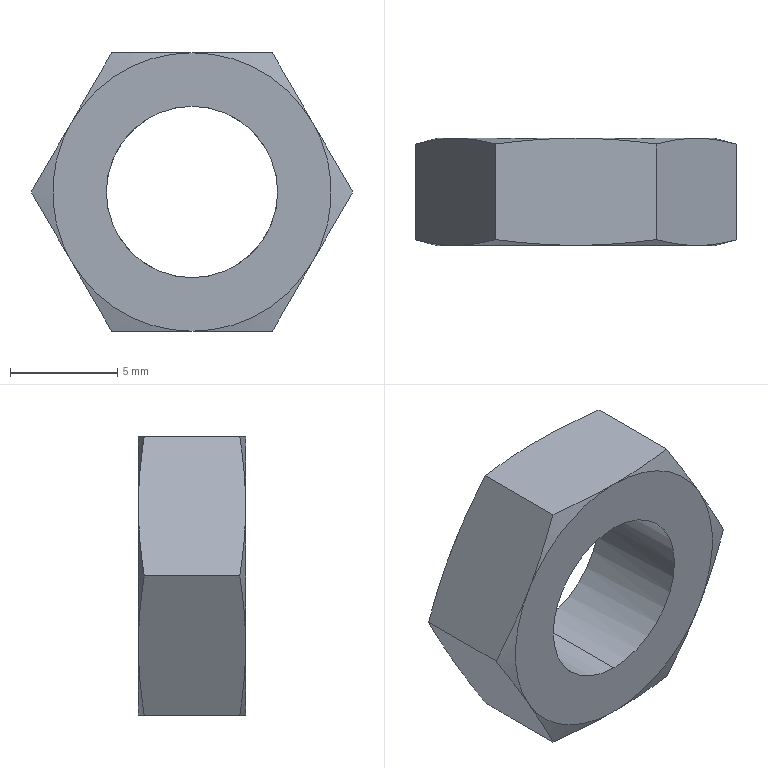Component | SolidWorks | HandlingMechanism-2_CDU25-40A-A93(0_0)-2_4..050.63-1 | 1 solid | 22 faces | box 15.01 x 5 x 13 mm | volume 478 mm3 | cone 12 | plane 8 | cylinder 2 | commonest cylinder face diameters 8 x2
STEP:
#1=CARTESIAN_POINT('',(1.019,4.705,5.787));
#2=VERTEX_POINT('',#1);
#3=CARTESIAN_POINT('',(1.019,4.705,6.102));
#4=VERTEX_POINT('',#3);
#5=CARTESIAN_POINT('',(1.019,4.705,5.945));
#6=DIRECTION('',(0.,1.,-0.));
#7=DIRECTION('',(0.,0.,1.));
#8=AXIS2_PLACEMENT_3D('',#5,#6,#7);
#9=CIRCLE('',#8,0.1575);
#10=EDGE_CURVE('',#2,#4,#9,.T.);
#11=ORIENTED_EDGE('',*,*,#10,.F.);
#12=CARTESIAN_POINT('',(1.019,4.902,5.787));
#13=VERTEX_POINT('',#12);
#14=CARTESIAN_POINT('',(1.019,4.705,5.787));
#15=DIRECTION('',(0.,1.,-0.));
#16=VECTOR('',#15,39.37);
#17=LINE('',#14,#16);
#18=EDGE_CURVE('',#2,#13,#17,.T.);
#19=ORIENTED_EDGE('',*,*,#18,.T.);
#20=CARTESIAN_POINT('',(1.019,4.902,6.102));
#21=VERTEX_POINT('',#20);
#22=CARTESIAN_POINT('',(1.019,4.902,5.787));
#23=CARTESIAN_POINT('',(0.9983,4.902,5.787));
#24=CARTESIAN_POINT('',(0.9777,4.902,5.792));
#25=CARTESIAN_POINT('',(0.9396,4.902,5.807));
#26=CARTESIAN_POINT('',(0.9221,4.902,5.819));
#27=CARTESIAN_POINT('',(0.893,4.902,5.848));
#28=CARTESIAN_POINT('',(0.8813,4.902,5.866));
#29=CARTESIAN_POINT('',(0.8655,4.902,5.904));
#30=CARTESIAN_POINT('',(0.8614,4.902,5.924));
#31=CARTESIAN_POINT('',(0.8614,4.902,5.965));
#32=CARTESIAN_POINT('',(0.8655,4.902,5.986));
#33=CARTESIAN_POINT('',(0.8813,4.902,6.024));
#34=CARTESIAN_POINT('',(0.893,4.902,6.042));
#35=CARTESIAN_POINT('',(0.9221,4.902,6.071));
#36=CARTESIAN_POINT('',(0.9396,4.902,6.082));
#37=CARTESIAN_POINT('',(0.9777,4.902,6.098));
#38=CARTESIAN_POINT('',(0.9983,4.902,6.102));
#39=CARTESIAN_POINT('',(1.019,4.902,6.102));
#40=B_SPLINE_CURVE_WITH_KNOTS('',3,(#22,#23,#24,#25,#26,#27,#28,#29,#30,#31,#32,#33,#34,#35,#36,#37,#38,#39),.UNSPECIFIED.,.F.,.F.,(4,2,2,2,2,2,2,2,4),(0.5,0.5625,0.625,0.6875,0.75,0.8125,0.875,0.9375,1.),.UNSPECIFIED.);
#41=EDGE_CURVE('',#13,#21,#40,.T.);
#42=ORIENTED_EDGE('',*,*,#41,.T.);
#43=CARTESIAN_POINT('',(1.019,4.705,6.102));
#44=DIRECTION('',(0.,1.,-0.));
#45=VECTOR('',#44,39.37);
#46=LINE('',#43,#45);
#47=EDGE_CURVE('',#4,#21,#46,.T.);
#48=ORIENTED_EDGE('',*,*,#47,.F.);
#49=EDGE_LOOP('',(#11,#19,#42,#48));
#50=FACE_OUTER_BOUND('',#49,.T.);
#51=CARTESIAN_POINT('',(1.019,4.705,5.945));
#52=DIRECTION('',(0.,1.,-0.));
#53=DIRECTION('',(0.,0.,1.));
#54=AXIS2_PLACEMENT_3D('',#51,#52,#53);
#55=CYLINDRICAL_SURFACE('',#54,0.1575);
#56=ADVANCED_FACE('',(#50),#55,.F.);
#57=CARTESIAN_POINT('',(1.019,4.705,5.945));
#58=DIRECTION('',(0.,1.,-0.));
#59=DIRECTION('',(0.,0.,1.));
#60=AXIS2_PLACEMENT_3D('',#57,#58,#59);
#61=CIRCLE('',#60,0.1575);
#62=EDGE_CURVE('',#4,#2,#61,.T.);
#63=ORIENTED_EDGE('',*,*,#62,.T.);
#64=ORIENTED_EDGE('',*,*,#10,.T.);
#65=EDGE_LOOP('',(#63,#64));
#66=FACE_BOUND('',#65,.T.);
#67=CARTESIAN_POINT('',(1.019,4.705,5.689));
#68=VERTEX_POINT('',#67);
#69=CARTESIAN_POINT('',(1.241,4.705,5.817));
#70=VERTEX_POINT('',#69);
#71=CARTESIAN_POINT('',(1.019,4.705,5.945));
#72=DIRECTION('',(-0.,-1.,0.));
#73=DIRECTION('',(0.,0.,1.));
#74=AXIS2_PLACEMENT_3D('',#71,#72,#73);
#75=CIRCLE('',#74,0.2559);
#76=EDGE_CURVE('',#68,#70,#75,.T.);
#77=ORIENTED_EDGE('',*,*,#76,.T.);
#78=CARTESIAN_POINT('',(1.241,4.705,6.073));
#79=VERTEX_POINT('',#78);
#80=CARTESIAN_POINT('',(1.019,4.705,5.945));
#81=DIRECTION('',(-0.,-1.,0.));
#82=DIRECTION('',(-0.,0.,1.));
#83=AXIS2_PLACEMENT_3D('',#80,#81,#82);
#84=CIRCLE('',#83,0.2559);
#85=EDGE_CURVE('',#70,#79,#84,.T.);
#86=ORIENTED_EDGE('',*,*,#85,.T.);
#87=CARTESIAN_POINT('',(1.019,4.705,6.201));
#88=VERTEX_POINT('',#87);
#89=CARTESIAN_POINT('',(1.019,4.705,5.945));
#90=DIRECTION('',(-0.,-1.,0.));
#91=DIRECTION('',(0.,0.,1.));
#92=AXIS2_PLACEMENT_3D('',#89,#90,#91);
#93=CIRCLE('',#92,0.2559);
#94=EDGE_CURVE('',#79,#88,#93,.T.);
#95=ORIENTED_EDGE('',*,*,#94,.T.);
#96=CARTESIAN_POINT('',(0.7973,4.705,6.073));
#97=VERTEX_POINT('',#96);
#98=CARTESIAN_POINT('',(1.019,4.705,5.945));
#99=DIRECTION('',(-0.,-1.,0.));
#100=DIRECTION('',(0.,0.,1.));
#101=AXIS2_PLACEMENT_3D('',#98,#99,#100);
#102=CIRCLE('',#101,0.2559);
#103=EDGE_CURVE('',#88,#97,#102,.T.);
#104=ORIENTED_EDGE('',*,*,#103,.T.);
#105=CARTESIAN_POINT('',(0.7973,4.705,5.817));
#106=VERTEX_POINT('',#105);
#107=CARTESIAN_POINT('',(1.019,4.705,5.945));
#108=DIRECTION('',(-0.,-1.,0.));
#109=DIRECTION('',(-0.,0.,1.));
#110=AXIS2_PLACEMENT_3D('',#107,#108,#109);
#111=CIRCLE('',#110,0.2559);
#112=EDGE_CURVE('',#97,#106,#111,.T.);
#113=ORIENTED_EDGE('',*,*,#112,.T.);
#114=CARTESIAN_POINT('',(1.019,4.705,5.945));
#115=DIRECTION('',(-0.,-1.,0.));
#116=DIRECTION('',(0.,0.,1.));
#117=AXIS2_PLACEMENT_3D('',#114,#115,#116);
#118=CIRCLE('',#117,0.2559);
#119=EDGE_CURVE('',#106,#68,#118,.T.);
#120=ORIENTED_EDGE('',*,*,#119,.T.);
#121=EDGE_LOOP('',(#77,#86,#95,#104,#113,#120));
#122=FACE_OUTER_BOUND('',#121,.T.);
#123=CARTESIAN_POINT('',(1.226,4.705,5.945));
#124=DIRECTION('',(-0.,-1.,-0.));
#125=DIRECTION('',(-0.,0.,-1.));
#126=AXIS2_PLACEMENT_3D('',#123,#124,#125);
#127=PLANE('',#126);
#128=ADVANCED_FACE('',(#66,#122),#127,.T.);
#129=ORIENTED_EDGE('',*,*,#85,.F.);
#130=CARTESIAN_POINT('',(1.314,4.715,5.945));
#131=VERTEX_POINT('',#130);
#132=CARTESIAN_POINT('',(1.241,4.705,5.817));
#133=CARTESIAN_POINT('',(1.265,4.705,5.86));
#134=CARTESIAN_POINT('',(1.29,4.709,5.902));
#135=CARTESIAN_POINT('',(1.314,4.715,5.945));
#136=B_SPLINE_CURVE_WITH_KNOTS('',3,(#132,#133,#134,#135),.UNSPECIFIED.,.F.,.F.,(4,4),(0.,0.003762),.UNSPECIFIED.);
#137=EDGE_CURVE('',#70,#131,#136,.T.);
#138=ORIENTED_EDGE('',*,*,#137,.T.);
#139=CARTESIAN_POINT('',(1.314,4.715,5.945));
#140=CARTESIAN_POINT('',(1.29,4.709,5.987));
#141=CARTESIAN_POINT('',(1.265,4.705,6.03));
#142=CARTESIAN_POINT('',(1.241,4.705,6.073));
#143=B_SPLINE_CURVE_WITH_KNOTS('',3,(#139,#140,#141,#142),.UNSPECIFIED.,.F.,.F.,(4,4),(0.,0.003762),.UNSPECIFIED.);
#144=EDGE_CURVE('',#131,#79,#143,.T.);
#145=ORIENTED_EDGE('',*,*,#144,.T.);
#146=EDGE_LOOP('',(#129,#138,#145));
#147=FACE_OUTER_BOUND('',#146,.T.);
#148=CARTESIAN_POINT('',(1.019,4.715,5.945));
#149=DIRECTION('',(0.,1.,-0.));
#150=DIRECTION('',(0.,0.,1.));
#151=AXIS2_PLACEMENT_3D('',#148,#149,#150);
#152=CONICAL_SURFACE('',#151,0.2957,1.309);
#153=ADVANCED_FACE('',(#147),#152,.T.);
#154=CARTESIAN_POINT('',(1.167,4.715,5.689));
#155=VERTEX_POINT('',#154);
#156=CARTESIAN_POINT('',(1.167,4.715,5.689));
#157=CARTESIAN_POINT('',(1.191,4.709,5.731));
#158=CARTESIAN_POINT('',(1.216,4.705,5.774));
#159=CARTESIAN_POINT('',(1.241,4.705,5.817));
#160=B_SPLINE_CURVE_WITH_KNOTS('',3,(#156,#157,#158,#159),.UNSPECIFIED.,.F.,.F.,(4,4),(0.,0.003762),.UNSPECIFIED.);
#161=EDGE_CURVE('',#155,#70,#160,.T.);
#162=ORIENTED_EDGE('',*,*,#161,.T.);
#163=ORIENTED_EDGE('',*,*,#76,.F.);
#164=CARTESIAN_POINT('',(1.019,4.705,5.689));
#165=CARTESIAN_POINT('',(1.068,4.705,5.689));
#166=CARTESIAN_POINT('',(1.118,4.709,5.689));
#167=CARTESIAN_POINT('',(1.167,4.715,5.689));
#168=B_SPLINE_CURVE_WITH_KNOTS('',3,(#164,#165,#166,#167),.UNSPECIFIED.,.F.,.F.,(4,4),(0.,0.003762),.UNSPECIFIED.);
#169=EDGE_CURVE('',#68,#155,#168,.T.);
#170=ORIENTED_EDGE('',*,*,#169,.T.);
#171=EDGE_LOOP('',(#162,#163,#170));
#172=FACE_OUTER_BOUND('',#171,.T.);
#173=CARTESIAN_POINT('',(1.019,4.715,5.945));
#174=DIRECTION('',(0.,1.,-0.));
#175=DIRECTION('',(0.,0.,1.));
#176=AXIS2_PLACEMENT_3D('',#173,#174,#175);
#177=CONICAL_SURFACE('',#176,0.2957,1.309);
#178=ADVANCED_FACE('',(#172),#177,.T.);
#179=CARTESIAN_POINT('',(0.8712,4.715,5.689));
#180=VERTEX_POINT('',#179);
#181=CARTESIAN_POINT('',(0.8712,4.715,5.689));
#182=CARTESIAN_POINT('',(0.9202,4.709,5.689));
#183=CARTESIAN_POINT('',(0.9694,4.705,5.689));
#184=CARTESIAN_POINT('',(1.019,4.705,5.689));
#185=B_SPLINE_CURVE_WITH_KNOTS('',3,(#181,#182,#183,#184),.UNSPECIFIED.,.F.,.F.,(4,4),(0.,0.003762),.UNSPECIFIED.);
#186=EDGE_CURVE('',#180,#68,#185,.T.);
#187=ORIENTED_EDGE('',*,*,#186,.T.);
#188=ORIENTED_EDGE('',*,*,#119,.F.);
#189=CARTESIAN_POINT('',(0.7973,4.705,5.817));
#190=CARTESIAN_POINT('',(0.822,4.705,5.774));
#191=CARTESIAN_POINT('',(0.8467,4.709,5.731));
#192=CARTESIAN_POINT('',(0.8712,4.715,5.689));
#193=B_SPLINE_CURVE_WITH_KNOTS('',3,(#189,#190,#191,#192),.UNSPECIFIED.,.F.,.F.,(4,4),(0.,0.003762),.UNSPECIFIED.);
#194=EDGE_CURVE('',#106,#180,#193,.T.);
#195=ORIENTED_EDGE('',*,*,#194,.T.);
#196=EDGE_LOOP('',(#187,#188,#195));
#197=FACE_OUTER_BOUND('',#196,.T.);
#198=CARTESIAN_POINT('',(1.019,4.715,5.945));
#199=DIRECTION('',(0.,1.,-0.));
#200=DIRECTION('',(0.,0.,1.));
#201=AXIS2_PLACEMENT_3D('',#198,#199,#200);
#202=CONICAL_SURFACE('',#201,0.2957,1.309);
#203=ADVANCED_FACE('',(#197),#202,.T.);
#204=CARTESIAN_POINT('',(0.7234,4.715,5.945));
#205=VERTEX_POINT('',#204);
#206=CARTESIAN_POINT('',(0.7234,4.715,5.945));
#207=CARTESIAN_POINT('',(0.7479,4.709,5.902));
#208=CARTESIAN_POINT('',(0.7725,4.705,5.86));
#209=CARTESIAN_POINT('',(0.7973,4.705,5.817));
#210=B_SPLINE_CURVE_WITH_KNOTS('',3,(#206,#207,#208,#209),.UNSPECIFIED.,.F.,.F.,(4,4),(0.,0.003762),.UNSPECIFIED.);
#211=EDGE_CURVE('',#205,#106,#210,.T.);
#212=ORIENTED_EDGE('',*,*,#211,.T.);
#213=ORIENTED_EDGE('',*,*,#112,.F.);
#214=CARTESIAN_POINT('',(0.7973,4.705,6.073));
#215=CARTESIAN_POINT('',(0.7725,4.705,6.03));
#216=CARTESIAN_POINT('',(0.7479,4.709,5.987));
#217=CARTESIAN_POINT('',(0.7234,4.715,5.945));
#218=B_SPLINE_CURVE_WITH_KNOTS('',3,(#214,#215,#216,#217),.UNSPECIFIED.,.F.,.F.,(4,4),(0.,0.003762),.UNSPECIFIED.);
#219=EDGE_CURVE('',#97,#205,#218,.T.);
#220=ORIENTED_EDGE('',*,*,#219,.T.);
#221=EDGE_LOOP('',(#212,#213,#220));
#222=FACE_OUTER_BOUND('',#221,.T.);
#223=CARTESIAN_POINT('',(1.019,4.715,5.945));
#224=DIRECTION('',(0.,1.,-0.));
#225=DIRECTION('',(0.,0.,1.));
#226=AXIS2_PLACEMENT_3D('',#223,#224,#225);
#227=CONICAL_SURFACE('',#226,0.2957,1.309);
#228=ADVANCED_FACE('',(#222),#227,.T.);
#229=ORIENTED_EDGE('',*,*,#103,.F.);
#230=CARTESIAN_POINT('',(0.8712,4.715,6.201));
#231=VERTEX_POINT('',#230);
#232=CARTESIAN_POINT('',(1.019,4.705,6.201));
#233=CARTESIAN_POINT('',(0.9694,4.705,6.201));
#234=CARTESIAN_POINT('',(0.9202,4.709,6.201));
#235=CARTESIAN_POINT('',(0.8712,4.715,6.201));
#236=B_SPLINE_CURVE_WITH_KNOTS('',3,(#232,#233,#234,#235),.UNSPECIFIED.,.F.,.F.,(4,4),(0.,0.003762),.UNSPECIFIED.);
#237=EDGE_CURVE('',#88,#231,#236,.T.);
#238=ORIENTED_EDGE('',*,*,#237,.T.);
#239=CARTESIAN_POINT('',(0.8712,4.715,6.201));
#240=CARTESIAN_POINT('',(0.8467,4.709,6.158));
#241=CARTESIAN_POINT('',(0.822,4.705,6.116));
#242=CARTESIAN_POINT('',(0.7973,4.705,6.073));
#243=B_SPLINE_CURVE_WITH_KNOTS('',3,(#239,#240,#241,#242),.UNSPECIFIED.,.F.,.F.,(4,4),(0.,0.003762),.UNSPECIFIED.);
#244=EDGE_CURVE('',#231,#97,#243,.T.);
#245=ORIENTED_EDGE('',*,*,#244,.T.);
#246=EDGE_LOOP('',(#229,#238,#245));
#247=FACE_OUTER_BOUND('',#246,.T.);
#248=CARTESIAN_POINT('',(1.019,4.715,5.945));
#249=DIRECTION('',(0.,1.,-0.));
#250=DIRECTION('',(0.,0.,1.));
#251=AXIS2_PLACEMENT_3D('',#248,#249,#250);
#252=CONICAL_SURFACE('',#251,0.2957,1.309);
#253=ADVANCED_FACE('',(#247),#252,.T.);
#254=ORIENTED_EDGE('',*,*,#94,.F.);
#255=CARTESIAN_POINT('',(1.167,4.715,6.201));
#256=VERTEX_POINT('',#255);
#257=CARTESIAN_POINT('',(1.241,4.705,6.073));
#258=CARTESIAN_POINT('',(1.216,4.705,6.116));
#259=CARTESIAN_POINT('',(1.191,4.709,6.158));
#260=CARTESIAN_POINT('',(1.167,4.715,6.201));
#261=B_SPLINE_CURVE_WITH_KNOTS('',3,(#257,#258,#259,#260),.UNSPECIFIED.,.F.,.F.,(4,4),(0.,0.003762),.UNSPECIFIED.);
#262=EDGE_CURVE('',#79,#256,#261,.T.);
#263=ORIENTED_EDGE('',*,*,#262,.T.);
#264=CARTESIAN_POINT('',(1.167,4.715,6.201));
#265=CARTESIAN_POINT('',(1.118,4.709,6.201));
#266=CARTESIAN_POINT('',(1.068,4.705,6.201));
#267=CARTESIAN_POINT('',(1.019,4.705,6.201));
#268=B_SPLINE_CURVE_WITH_KNOTS('',3,(#264,#265,#266,#267),.UNSPECIFIED.,.F.,.F.,(4,4),(0.,0.003762),.UNSPECIFIED.);
#269=EDGE_CURVE('',#256,#88,#268,.T.);
#270=ORIENTED_EDGE('',*,*,#269,.T.);
#271=EDGE_LOOP('',(#254,#263,#270));
#272=FACE_OUTER_BOUND('',#271,.T.);
#273=CARTESIAN_POINT('',(1.019,4.715,5.945));
#274=DIRECTION('',(0.,1.,-0.));
#275=DIRECTION('',(0.,0.,1.));
#276=AXIS2_PLACEMENT_3D('',#273,#274,#275);
#277=CONICAL_SURFACE('',#276,0.2957,1.309);
#278=ADVANCED_FACE('',(#272),#277,.T.);
#279=CARTESIAN_POINT('',(1.167,4.891,5.689));
#280=VERTEX_POINT('',#279);
#281=CARTESIAN_POINT('',(1.167,4.902,5.689));
#282=DIRECTION('',(-0.,-1.,0.));
#283=VECTOR('',#282,39.37);
#284=LINE('',#281,#283);
#285=EDGE_CURVE('',#280,#155,#284,.T.);
#286=ORIENTED_EDGE('',*,*,#285,.F.);
#287=CARTESIAN_POINT('',(1.241,4.902,5.817));
#288=VERTEX_POINT('',#287);
#289=CARTESIAN_POINT('',(1.241,4.902,5.817));
#290=CARTESIAN_POINT('',(1.216,4.902,5.774));
#291=CARTESIAN_POINT('',(1.191,4.898,5.731));
#292=CARTESIAN_POINT('',(1.167,4.891,5.689));
#293=B_SPLINE_CURVE_WITH_KNOTS('',3,(#289,#290,#291,#292),.UNSPECIFIED.,.F.,.F.,(4,4),(0.,0.003762),.UNSPECIFIED.);
#294=EDGE_CURVE('',#288,#280,#293,.T.);
#295=ORIENTED_EDGE('',*,*,#294,.F.);
#296=CARTESIAN_POINT('',(1.314,4.891,5.945));
#297=VERTEX_POINT('',#296);
#298=CARTESIAN_POINT('',(1.314,4.891,5.945));
#299=CARTESIAN_POINT('',(1.29,4.898,5.902));
#300=CARTESIAN_POINT('',(1.265,4.902,5.86));
#301=CARTESIAN_POINT('',(1.241,4.902,5.817));
#302=B_SPLINE_CURVE_WITH_KNOTS('',3,(#298,#299,#300,#301),.UNSPECIFIED.,.F.,.F.,(4,4),(0.,0.003762),.UNSPECIFIED.);
#303=EDGE_CURVE('',#297,#288,#302,.T.);
#304=ORIENTED_EDGE('',*,*,#303,.F.);
#305=CARTESIAN_POINT('',(1.314,4.902,5.945));
#306=DIRECTION('',(0.,1.,-0.));
#307=VECTOR('',#306,39.37);
#308=LINE('',#305,#307);
#309=EDGE_CURVE('',#131,#297,#308,.T.);
#310=ORIENTED_EDGE('',*,*,#309,.F.);
#311=ORIENTED_EDGE('',*,*,#137,.F.);
#312=ORIENTED_EDGE('',*,*,#161,.F.);
#313=EDGE_LOOP('',(#286,#295,#304,#310,#311,#312));
#314=FACE_OUTER_BOUND('',#313,.T.);
#315=CARTESIAN_POINT('',(1.167,4.902,5.689));
#316=DIRECTION('',(-0.866,0.,0.5));
#317=DIRECTION('',(0.5,-0.,0.866));
#318=AXIS2_PLACEMENT_3D('',#315,#316,#317);
#319=PLANE('',#318);
#320=ADVANCED_FACE('',(#314),#319,.F.);
#321=CARTESIAN_POINT('',(0.8712,4.891,5.689));
#322=VERTEX_POINT('',#321);
#323=CARTESIAN_POINT('',(0.8712,4.902,5.689));
#324=DIRECTION('',(-0.,-1.,0.));
#325=VECTOR('',#324,39.37);
#326=LINE('',#323,#325);
#327=EDGE_CURVE('',#322,#180,#326,.T.);
#328=ORIENTED_EDGE('',*,*,#327,.F.);
#329=CARTESIAN_POINT('',(1.019,4.902,5.689));
#330=VERTEX_POINT('',#329);
#331=CARTESIAN_POINT('',(1.019,4.902,5.689));
#332=CARTESIAN_POINT('',(0.9694,4.902,5.689));
#333=CARTESIAN_POINT('',(0.9202,4.898,5.689));
#334=CARTESIAN_POINT('',(0.8712,4.891,5.689));
#335=B_SPLINE_CURVE_WITH_KNOTS('',3,(#331,#332,#333,#334),.UNSPECIFIED.,.F.,.F.,(4,4),(0.,0.003762),.UNSPECIFIED.);
#336=EDGE_CURVE('',#330,#322,#335,.T.);
#337=ORIENTED_EDGE('',*,*,#336,.F.);
#338=CARTESIAN_POINT('',(1.167,4.891,5.689));
#339=CARTESIAN_POINT('',(1.118,4.898,5.689));
#340=CARTESIAN_POINT('',(1.068,4.902,5.689));
#341=CARTESIAN_POINT('',(1.019,4.902,5.689));
#342=B_SPLINE_CURVE_WITH_KNOTS('',3,(#338,#339,#340,#341),.UNSPECIFIED.,.F.,.F.,(4,4),(0.,0.003762),.UNSPECIFIED.);
#343=EDGE_CURVE('',#280,#330,#342,.T.);
#344=ORIENTED_EDGE('',*,*,#343,.F.);
#345=ORIENTED_EDGE('',*,*,#285,.T.);
#346=ORIENTED_EDGE('',*,*,#169,.F.);
#347=ORIENTED_EDGE('',*,*,#186,.F.);
#348=EDGE_LOOP('',(#328,#337,#344,#345,#346,#347));
#349=FACE_OUTER_BOUND('',#348,.T.);
#350=CARTESIAN_POINT('',(0.8712,4.902,5.689));
#351=DIRECTION('',(0.,0.,1.));
#352=DIRECTION('',(-0.,-1.,0.));
#353=AXIS2_PLACEMENT_3D('',#350,#351,#352);
#354=PLANE('',#353);
#355=ADVANCED_FACE('',(#349),#354,.F.);
#356=CARTESIAN_POINT('',(0.7234,4.891,5.945));
#357=VERTEX_POINT('',#356);
#358=CARTESIAN_POINT('',(0.7234,4.902,5.945));
#359=DIRECTION('',(-0.,-1.,0.));
#360=VECTOR('',#359,39.37);
#361=LINE('',#358,#360);
#362=EDGE_CURVE('',#357,#205,#361,.T.);
#363=ORIENTED_EDGE('',*,*,#362,.F.);
#364=CARTESIAN_POINT('',(0.7973,4.902,5.817));
#365=VERTEX_POINT('',#364);
#366=CARTESIAN_POINT('',(0.7973,4.902,5.817));
#367=CARTESIAN_POINT('',(0.7725,4.902,5.86));
#368=CARTESIAN_POINT('',(0.7479,4.898,5.902));
#369=CARTESIAN_POINT('',(0.7234,4.891,5.945));
#370=B_SPLINE_CURVE_WITH_KNOTS('',3,(#366,#367,#368,#369),.UNSPECIFIED.,.F.,.F.,(4,4),(0.,0.003762),.UNSPECIFIED.);
#371=EDGE_CURVE('',#365,#357,#370,.T.);
#372=ORIENTED_EDGE('',*,*,#371,.F.);
#373=CARTESIAN_POINT('',(0.8712,4.891,5.689));
#374=CARTESIAN_POINT('',(0.8467,4.898,5.731));
#375=CARTESIAN_POINT('',(0.822,4.902,5.774));
#376=CARTESIAN_POINT('',(0.7973,4.902,5.817));
#377=B_SPLINE_CURVE_WITH_KNOTS('',3,(#373,#374,#375,#376),.UNSPECIFIED.,.F.,.F.,(4,4),(0.,0.003762),.UNSPECIFIED.);
#378=EDGE_CURVE('',#322,#365,#377,.T.);
#379=ORIENTED_EDGE('',*,*,#378,.F.);
#380=ORIENTED_EDGE('',*,*,#327,.T.);
#381=ORIENTED_EDGE('',*,*,#194,.F.);
#382=ORIENTED_EDGE('',*,*,#211,.F.);
#383=EDGE_LOOP('',(#363,#372,#379,#380,#381,#382));
#384=FACE_OUTER_BOUND('',#383,.T.);
#385=CARTESIAN_POINT('',(0.7234,4.902,5.945));
#386=DIRECTION('',(0.866,-0.,0.5));
#387=DIRECTION('',(0.5,-0.,-0.866));
#388=AXIS2_PLACEMENT_3D('',#385,#386,#387);
#389=PLANE('',#388);
#390=ADVANCED_FACE('',(#384),#389,.F.);
#391=ORIENTED_EDGE('',*,*,#244,.F.);
#392=CARTESIAN_POINT('',(0.8712,4.891,6.201));
#393=VERTEX_POINT('',#392);
#394=CARTESIAN_POINT('',(0.8712,4.902,6.201));
#395=DIRECTION('',(-0.,-1.,0.));
#396=VECTOR('',#395,39.37);
#397=LINE('',#394,#396);
#398=EDGE_CURVE('',#393,#231,#397,.T.);
#399=ORIENTED_EDGE('',*,*,#398,.F.);
#400=CARTESIAN_POINT('',(0.7973,4.902,6.073));
#401=VERTEX_POINT('',#400);
#402=CARTESIAN_POINT('',(0.7973,4.902,6.073));
#403=CARTESIAN_POINT('',(0.822,4.902,6.116));
#404=CARTESIAN_POINT('',(0.8467,4.898,6.158));
#405=CARTESIAN_POINT('',(0.8712,4.891,6.201));
#406=B_SPLINE_CURVE_WITH_KNOTS('',3,(#402,#403,#404,#405),.UNSPECIFIED.,.F.,.F.,(4,4),(0.,0.003762),.UNSPECIFIED.);
#407=EDGE_CURVE('',#401,#393,#406,.T.);
#408=ORIENTED_EDGE('',*,*,#407,.F.);
#409=CARTESIAN_POINT('',(0.7234,4.891,5.945));
#410=CARTESIAN_POINT('',(0.7479,4.898,5.987));
#411=CARTESIAN_POINT('',(0.7725,4.902,6.03));
#412=CARTESIAN_POINT('',(0.7973,4.902,6.073));
#413=B_SPLINE_CURVE_WITH_KNOTS('',3,(#409,#410,#411,#412),.UNSPECIFIED.,.F.,.F.,(4,4),(0.,0.003762),.UNSPECIFIED.);
#414=EDGE_CURVE('',#357,#401,#413,.T.);
#415=ORIENTED_EDGE('',*,*,#414,.F.);
#416=ORIENTED_EDGE('',*,*,#362,.T.);
#417=ORIENTED_EDGE('',*,*,#219,.F.);
#418=EDGE_LOOP('',(#391,#399,#408,#415,#416,#417));
#419=FACE_OUTER_BOUND('',#418,.T.);
#420=CARTESIAN_POINT('',(0.8712,4.902,6.201));
#421=DIRECTION('',(0.866,-0.,-0.5));
#422=DIRECTION('',(-0.5,0.,-0.866));
#423=AXIS2_PLACEMENT_3D('',#420,#421,#422);
#424=PLANE('',#423);
#425=ADVANCED_FACE('',(#419),#424,.F.);
#426=ORIENTED_EDGE('',*,*,#269,.F.);
#427=CARTESIAN_POINT('',(1.167,4.891,6.201));
#428=VERTEX_POINT('',#427);
#429=CARTESIAN_POINT('',(1.167,4.902,6.201));
#430=DIRECTION('',(-0.,-1.,0.));
#431=VECTOR('',#430,39.37);
#432=LINE('',#429,#431);
#433=EDGE_CURVE('',#428,#256,#432,.T.);
#434=ORIENTED_EDGE('',*,*,#433,.F.);
#435=CARTESIAN_POINT('',(1.019,4.902,6.201));
#436=VERTEX_POINT('',#435);
#437=CARTESIAN_POINT('',(1.019,4.902,6.201));
#438=CARTESIAN_POINT('',(1.068,4.902,6.201));
#439=CARTESIAN_POINT('',(1.118,4.898,6.201));
#440=CARTESIAN_POINT('',(1.167,4.891,6.201));
#441=B_SPLINE_CURVE_WITH_KNOTS('',3,(#437,#438,#439,#440),.UNSPECIFIED.,.F.,.F.,(4,4),(0.,0.003762),.UNSPECIFIED.);
#442=EDGE_CURVE('',#436,#428,#441,.T.);
#443=ORIENTED_EDGE('',*,*,#442,.F.);
#444=CARTESIAN_POINT('',(0.8712,4.891,6.201));
#445=CARTESIAN_POINT('',(0.9202,4.898,6.201));
#446=CARTESIAN_POINT('',(0.9694,4.902,6.201));
#447=CARTESIAN_POINT('',(1.019,4.902,6.201));
#448=B_SPLINE_CURVE_WITH_KNOTS('',3,(#444,#445,#446,#447),.UNSPECIFIED.,.F.,.F.,(4,4),(0.,0.003762),.UNSPECIFIED.);
#449=EDGE_CURVE('',#393,#436,#448,.T.);
#450=ORIENTED_EDGE('',*,*,#449,.F.);
#451=ORIENTED_EDGE('',*,*,#398,.T.);
#452=ORIENTED_EDGE('',*,*,#237,.F.);
#453=EDGE_LOOP('',(#426,#434,#443,#450,#451,#452));
#454=FACE_OUTER_BOUND('',#453,.T.);
#455=CARTESIAN_POINT('',(1.167,4.902,6.201));
#456=DIRECTION('',(-0.,-0.,-1.));
#457=DIRECTION('',(0.,1.,-0.));
#458=AXIS2_PLACEMENT_3D('',#455,#456,#457);
#459=PLANE('',#458);
#460=ADVANCED_FACE('',(#454),#459,.F.);
#461=ORIENTED_EDGE('',*,*,#144,.F.);
#462=ORIENTED_EDGE('',*,*,#309,.T.);
#463=CARTESIAN_POINT('',(1.241,4.902,6.073));
#464=VERTEX_POINT('',#463);
#465=CARTESIAN_POINT('',(1.241,4.902,6.073));
#466=CARTESIAN_POINT('',(1.265,4.902,6.03));
#467=CARTESIAN_POINT('',(1.29,4.898,5.987));
#468=CARTESIAN_POINT('',(1.314,4.891,5.945));
#469=B_SPLINE_CURVE_WITH_KNOTS('',3,(#465,#466,#467,#468),.UNSPECIFIED.,.F.,.F.,(4,4),(0.,0.003762),.UNSPECIFIED.);
#470=EDGE_CURVE('',#464,#297,#469,.T.);
#471=ORIENTED_EDGE('',*,*,#470,.F.);
#472=CARTESIAN_POINT('',(1.167,4.891,6.201));
#473=CARTESIAN_POINT('',(1.191,4.898,6.158));
#474=CARTESIAN_POINT('',(1.216,4.902,6.116));
#475=CARTESIAN_POINT('',(1.241,4.902,6.073));
#476=B_SPLINE_CURVE_WITH_KNOTS('',3,(#472,#473,#474,#475),.UNSPECIFIED.,.F.,.F.,(4,4),(0.,0.003762),.UNSPECIFIED.);
#477=EDGE_CURVE('',#428,#464,#476,.T.);
#478=ORIENTED_EDGE('',*,*,#477,.F.);
#479=ORIENTED_EDGE('',*,*,#433,.T.);
#480=ORIENTED_EDGE('',*,*,#262,.F.);
#481=EDGE_LOOP('',(#461,#462,#471,#478,#479,#480));
#482=FACE_OUTER_BOUND('',#481,.T.);
#483=CARTESIAN_POINT('',(1.314,4.902,5.945));
#484=DIRECTION('',(-0.866,0.,-0.5));
#485=DIRECTION('',(-0.5,0.,0.866));
#486=AXIS2_PLACEMENT_3D('',#483,#484,#485);
#487=PLANE('',#486);
#488=ADVANCED_FACE('',(#482),#487,.F.);
#489=ORIENTED_EDGE('',*,*,#343,.T.);
#490=CARTESIAN_POINT('',(1.019,4.902,5.945));
#491=DIRECTION('',(-0.,-1.,0.));
#492=DIRECTION('',(-0.,0.,-1.));
#493=AXIS2_PLACEMENT_3D('',#490,#491,#492);
#494=CIRCLE('',#493,0.2559);
#495=EDGE_CURVE('',#330,#288,#494,.T.);
#496=ORIENTED_EDGE('',*,*,#495,.T.);
#497=ORIENTED_EDGE('',*,*,#294,.T.);
#498=EDGE_LOOP('',(#489,#496,#497));
#499=FACE_OUTER_BOUND('',#498,.T.);
#500=CARTESIAN_POINT('',(1.019,4.891,5.945));
#501=DIRECTION('',(-0.,-1.,0.));
#502=DIRECTION('',(-0.,0.,-1.));
#503=AXIS2_PLACEMENT_3D('',#500,#501,#502);
#504=CONICAL_SURFACE('',#503,0.2957,1.309);
#505=ADVANCED_FACE('',(#499),#504,.T.);
#506=ORIENTED_EDGE('',*,*,#303,.T.);
#507=CARTESIAN_POINT('',(1.019,4.902,5.945));
#508=DIRECTION('',(-0.,-1.,0.));
#509=DIRECTION('',(-0.,0.,-1.));
#510=AXIS2_PLACEMENT_3D('',#507,#508,#509);
#511=CIRCLE('',#510,0.2559);
#512=EDGE_CURVE('',#288,#464,#511,.T.);
#513=ORIENTED_EDGE('',*,*,#512,.T.);
#514=ORIENTED_EDGE('',*,*,#470,.T.);
#515=EDGE_LOOP('',(#506,#513,#514));
#516=FACE_OUTER_BOUND('',#515,.T.);
#517=CARTESIAN_POINT('',(1.019,4.891,5.945));
#518=DIRECTION('',(-0.,-1.,0.));
#519=DIRECTION('',(-0.,0.,-1.));
#520=AXIS2_PLACEMENT_3D('',#517,#518,#519);
#521=CONICAL_SURFACE('',#520,0.2957,1.309);
#522=ADVANCED_FACE('',(#516),#521,.T.);
#523=CARTESIAN_POINT('',(1.019,4.902,5.945));
#524=DIRECTION('',(-0.,-1.,0.));
#525=DIRECTION('',(-0.,0.,-1.));
#526=AXIS2_PLACEMENT_3D('',#523,#524,#525);
#527=CIRCLE('',#526,0.2559);
#528=EDGE_CURVE('',#365,#330,#527,.T.);
#529=ORIENTED_EDGE('',*,*,#528,.T.);
#530=ORIENTED_EDGE('',*,*,#336,.T.);
#531=ORIENTED_EDGE('',*,*,#378,.T.);
#532=EDGE_LOOP('',(#529,#530,#531));
#533=FACE_OUTER_BOUND('',#532,.T.);
#534=CARTESIAN_POINT('',(1.019,4.891,5.945));
#535=DIRECTION('',(-0.,-1.,0.));
#536=DIRECTION('',(-0.,0.,-1.));
#537=AXIS2_PLACEMENT_3D('',#534,#535,#536);
#538=CONICAL_SURFACE('',#537,0.2957,1.309);
#539=ADVANCED_FACE('',(#533),#538,.T.);
#540=CARTESIAN_POINT('',(1.019,4.902,5.945));
#541=DIRECTION('',(-0.,-1.,0.));
#542=DIRECTION('',(-0.,0.,-1.));
#543=AXIS2_PLACEMENT_3D('',#540,#541,#542);
#544=CIRCLE('',#543,0.2559);
#545=EDGE_CURVE('',#401,#365,#544,.T.);
#546=ORIENTED_EDGE('',*,*,#545,.T.);
#547=ORIENTED_EDGE('',*,*,#371,.T.);
#548=ORIENTED_EDGE('',*,*,#414,.T.);
#549=EDGE_LOOP('',(#546,#547,#548));
#550=FACE_OUTER_BOUND('',#549,.T.);
#551=CARTESIAN_POINT('',(1.019,4.891,5.945));
#552=DIRECTION('',(-0.,-1.,0.));
#553=DIRECTION('',(-0.,0.,-1.));
#554=AXIS2_PLACEMENT_3D('',#551,#552,#553);
#555=CONICAL_SURFACE('',#554,0.2957,1.309);
#556=ADVANCED_FACE('',(#550),#555,.T.);
#557=CARTESIAN_POINT('',(1.019,4.902,5.945));
#558=DIRECTION('',(-0.,-1.,0.));
#559=DIRECTION('',(-0.,0.,-1.));
#560=AXIS2_PLACEMENT_3D('',#557,#558,#559);
#561=CIRCLE('',#560,0.2559);
#562=EDGE_CURVE('',#436,#401,#561,.T.);
#563=ORIENTED_EDGE('',*,*,#562,.T.);
#564=ORIENTED_EDGE('',*,*,#407,.T.);
#565=ORIENTED_EDGE('',*,*,#449,.T.);
#566=EDGE_LOOP('',(#563,#564,#565));
#567=FACE_OUTER_BOUND('',#566,.T.);
#568=CARTESIAN_POINT('',(1.019,4.891,5.945));
#569=DIRECTION('',(-0.,-1.,0.));
#570=DIRECTION('',(-0.,0.,-1.));
#571=AXIS2_PLACEMENT_3D('',#568,#569,#570);
#572=CONICAL_SURFACE('',#571,0.2957,1.309);
#573=ADVANCED_FACE('',(#567),#572,.T.);
#574=ORIENTED_EDGE('',*,*,#477,.T.);
#575=CARTESIAN_POINT('',(1.019,4.902,5.945));
#576=DIRECTION('',(-0.,-1.,0.));
#577=DIRECTION('',(-0.,0.,-1.));
#578=AXIS2_PLACEMENT_3D('',#575,#576,#577);
#579=CIRCLE('',#578,0.2559);
#580=EDGE_CURVE('',#464,#436,#579,.T.);
#581=ORIENTED_EDGE('',*,*,#580,.T.);
#582=ORIENTED_EDGE('',*,*,#442,.T.);
#583=EDGE_LOOP('',(#574,#581,#582));
#584=FACE_OUTER_BOUND('',#583,.T.);
#585=CARTESIAN_POINT('',(1.019,4.891,5.945));
#586=DIRECTION('',(-0.,-1.,0.));
#587=DIRECTION('',(-0.,0.,-1.));
#588=AXIS2_PLACEMENT_3D('',#585,#586,#587);
#589=CONICAL_SURFACE('',#588,0.2957,1.309);
#590=ADVANCED_FACE('',(#584),#589,.T.);
#591=ORIENTED_EDGE('',*,*,#562,.F.);
#592=ORIENTED_EDGE('',*,*,#580,.F.);
#593=ORIENTED_EDGE('',*,*,#512,.F.);
#594=ORIENTED_EDGE('',*,*,#495,.F.);
#595=ORIENTED_EDGE('',*,*,#528,.F.);
#596=ORIENTED_EDGE('',*,*,#545,.F.);
#597=EDGE_LOOP('',(#591,#592,#593,#594,#595,#596));
#598=FACE_OUTER_BOUND('',#597,.T.);
#599=CARTESIAN_POINT('',(1.019,4.902,6.102));
#600=CARTESIAN_POINT('',(1.04,4.902,6.102));
#601=CARTESIAN_POINT('',(1.06,4.902,6.098));
#602=CARTESIAN_POINT('',(1.098,4.902,6.082));
#603=CARTESIAN_POINT('',(1.116,4.902,6.071));
#604=CARTESIAN_POINT('',(1.145,4.902,6.042));
#605=CARTESIAN_POINT('',(1.157,4.902,6.024));
#606=CARTESIAN_POINT('',(1.172,4.902,5.986));
#607=CARTESIAN_POINT('',(1.176,4.902,5.965));
#608=CARTESIAN_POINT('',(1.176,4.902,5.924));
#609=CARTESIAN_POINT('',(1.172,4.902,5.904));
#610=CARTESIAN_POINT('',(1.157,4.902,5.866));
#611=CARTESIAN_POINT('',(1.145,4.902,5.848));
#612=CARTESIAN_POINT('',(1.116,4.902,5.819));
#613=CARTESIAN_POINT('',(1.098,4.902,5.807));
#614=CARTESIAN_POINT('',(1.06,4.902,5.792));
#615=CARTESIAN_POINT('',(1.04,4.902,5.787));
#616=CARTESIAN_POINT('',(1.019,4.902,5.787));
#617=B_SPLINE_CURVE_WITH_KNOTS('',3,(#599,#600,#601,#602,#603,#604,#605,#606,#607,#608,#609,#610,#611,#612,#613,#614,#615,#616),.UNSPECIFIED.,.F.,.F.,(4,2,2,2,2,2,2,2,4),(0.,0.0625,0.125,0.1875,0.25,0.3125,0.375,0.4375,0.5),.UNSPECIFIED.);
#618=EDGE_CURVE('',#21,#13,#617,.T.);
#619=ORIENTED_EDGE('',*,*,#618,.F.);
#620=ORIENTED_EDGE('',*,*,#41,.F.);
#621=EDGE_LOOP('',(#619,#620));
#622=FACE_BOUND('',#621,.T.);
#623=CARTESIAN_POINT('',(1.226,4.902,5.945));
#624=DIRECTION('',(0.,1.,0.));
#625=DIRECTION('',(0.,-0.,1.));
#626=AXIS2_PLACEMENT_3D('',#623,#624,#625);
#627=PLANE('',#626);
#628=ADVANCED_FACE('',(#598,#622),#627,.T.);
#629=ORIENTED_EDGE('',*,*,#18,.F.);
#630=ORIENTED_EDGE('',*,*,#62,.F.);
#631=ORIENTED_EDGE('',*,*,#47,.T.);
#632=ORIENTED_EDGE('',*,*,#618,.T.);
#633=EDGE_LOOP('',(#629,#630,#631,#632));
#634=FACE_OUTER_BOUND('',#633,.T.);
#635=CARTESIAN_POINT('',(1.019,4.705,5.945));
#636=DIRECTION('',(0.,1.,-0.));
#637=DIRECTION('',(0.,0.,1.));
#638=AXIS2_PLACEMENT_3D('',#635,#636,#637);
#639=CYLINDRICAL_SURFACE('',#638,0.1575);
#640=ADVANCED_FACE('',(#634),#639,.F.);
#641=CLOSED_SHELL('',(#56,#128,#153,#178,#203,#228,#253,#278,#320,#355,#390,#425,#460,#488,#505,#522,#539,#556,#573,#590,#628,#640));
#642=MANIFOLD_SOLID_BREP('',#641);
#643=CARTESIAN_POINT('',(0.,0.,0.));
#644=DIRECTION('',(0.,0.,1.));
#645=DIRECTION('',(1.,0.,0.));
#646=AXIS2_PLACEMENT_3D('',#643,#644,#645);
#647=(LENGTH_UNIT()NAMED_UNIT(*)SI_UNIT($,.METRE.));
#648=LENGTH_MEASURE_WITH_UNIT(LENGTH_MEASURE(0.0254),#647);
#649=DIMENSIONAL_EXPONENTS(1.,0.,0.,0.,0.,0.,0.);
#650=(CONVERSION_BASED_UNIT('',#648)LENGTH_UNIT()NAMED_UNIT(#649));
#651=UNCERTAINTY_MEASURE_WITH_UNIT(LENGTH_MEASURE(0.00001),#650,'','');
#652=(NAMED_UNIT(*)PLANE_ANGLE_UNIT()SI_UNIT($,.RADIAN.));
#653=(NAMED_UNIT(*)SI_UNIT($,.STERADIAN.)SOLID_ANGLE_UNIT());
#654=(GEOMETRIC_REPRESENTATION_CONTEXT(3)GLOBAL_UNCERTAINTY_ASSIGNED_CONTEXT((#651))GLOBAL_UNIT_ASSIGNED_CONTEXT((#650,#652,#653))REPRESENTATION_CONTEXT('',''));
#655=ADVANCED_BREP_SHAPE_REPRESENTATION('',(#642,#646),#654);
#656=COLOUR_RGB('',0.7922,0.8196,0.9333);
#657=FILL_AREA_STYLE_COLOUR('',#656);
#658=FILL_AREA_STYLE('',(#657));
#659=SURFACE_STYLE_FILL_AREA(#658);
#660=SURFACE_SIDE_STYLE('',(#659));
#661=SURFACE_STYLE_USAGE(.BOTH.,#660);
#662=PRESENTATION_STYLE_ASSIGNMENT((#661));
#663=STYLED_ITEM('',(#662),#642);
#664=(LENGTH_UNIT()NAMED_UNIT(*)SI_UNIT($,.METRE.));
#665=LENGTH_MEASURE_WITH_UNIT(LENGTH_MEASURE(0.0254),#664);
#666=DIMENSIONAL_EXPONENTS(1.,0.,0.,0.,0.,0.,0.);
#667=(CONVERSION_BASED_UNIT('',#665)LENGTH_UNIT()NAMED_UNIT(#666));
#668=UNCERTAINTY_MEASURE_WITH_UNIT(LENGTH_MEASURE(0.00001),#667,'','');
#669=(NAMED_UNIT(*)PLANE_ANGLE_UNIT()SI_UNIT($,.RADIAN.));
#670=(NAMED_UNIT(*)SI_UNIT($,.STERADIAN.)SOLID_ANGLE_UNIT());
#671=(GEOMETRIC_REPRESENTATION_CONTEXT(3)GLOBAL_UNCERTAINTY_ASSIGNED_CONTEXT((#668))GLOBAL_UNIT_ASSIGNED_CONTEXT((#667,#669,#670))REPRESENTATION_CONTEXT('',''));
#672=MECHANICAL_DESIGN_GEOMETRIC_PRESENTATION_REPRESENTATION('',(#663),#671);
#673=PRESENTATION_LAYER_ASSIGNMENT('','',(#663));